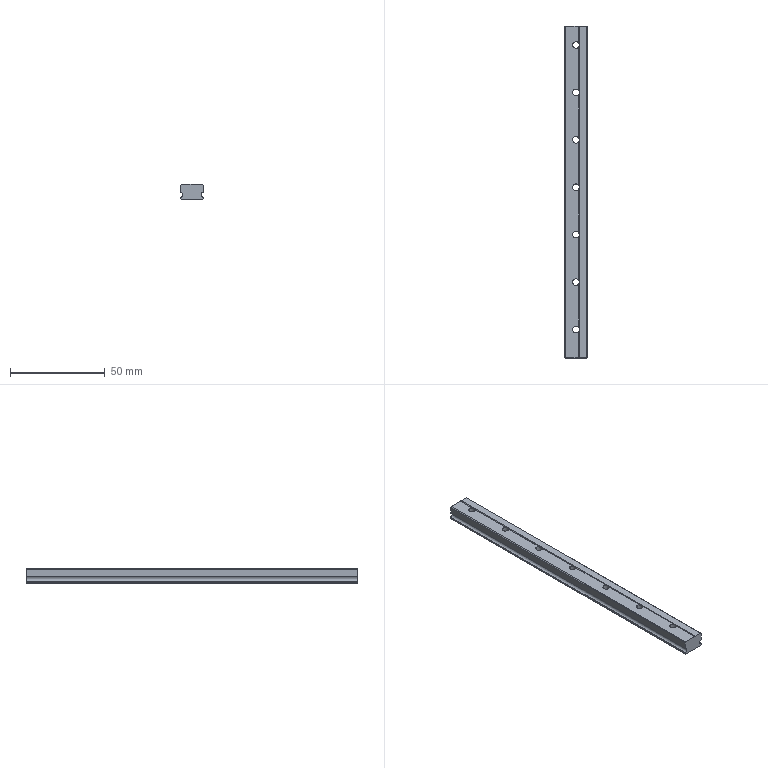Component | SolidWorks | MGN12H1R175Z0CGuideRailAssembly-1_MGN12HGuideRail-1 | 1 solid | 52 faces | box 12 x 175 x 8 mm | volume 14866 mm3 | cylinder 32 | plane 20 | commonest cylinder face diameters 6 x14 3.5 x14 2.5 x3 0.6 x1 | material 6061 Alloy
build123d program:
from build123d import *

# Parameters (mm, degrees)
SKETCH1_W                                            = 12
SKETCH1_H                                            = 175
BOSS_EXTRUDE1_DEPTH                                  = 8
F_2_5_2_5_DIAMETER_HOLE1_D                           = 2.5
F_0_6_0_6_DIAMETER_HOLE1_D                           = 0.6
CYLINDRICAL_COUNTERSUNK_HOLE_1_FOR_M3_HE_D           = 3.5
CYLINDRICAL_COUNTERSUNK_HOLE_1_FOR_M3_HE_CBORE_D     = 6
CYLINDRICAL_COUNTERSUNK_HOLE_1_FOR_M3_HE_CBORE_DEPTH = 3.5
CHAMFER1_SIZE                                        = 0.4
LPATTERN1_COUNT                                      = 7
LPATTERN1_PITCH                                      = 25


with BuildPart() as part:
    # Sketch1 → Boss-Extrude1 (new body)
    with BuildSketch(Plane.XZ):
        Rectangle(SKETCH1_W, SKETCH1_H)
    extrude(amount=-BOSS_EXTRUDE1_DEPTH)

    # 2.5 _2.5_ Diameter Hole1 (through all)
    with Locations(Plane(origin=(0, 0, -87.5), x_dir=(-1, 0, 0), z_dir=(0, 0, -1))):
        with Locations((-6, 5.5), (6, 5.5)):
            Hole(F_2_5_2_5_DIAMETER_HOLE1_D / 2)

    # 0.6 _0.6_ Diameter Hole1 (through all)
    with Locations(Plane.XY.offset(87.5)):
        with Locations((1.5, 0)):
            Hole(F_0_6_0_6_DIAMETER_HOLE1_D / 2)

    # Cylindrical Countersunk Hole 1 for M3 He (through all)
    with Locations(Plane(origin=(0, 8, 0), x_dir=(1, 0, 0), z_dir=(0, 1, 0))):
        with Locations((0, -77.5)):
            cylindrical_countersunk_hole_1_for_m3_he = CounterBoreHole(CYLINDRICAL_COUNTERSUNK_HOLE_1_FOR_M3_HE_D / 2, CYLINDRICAL_COUNTERSUNK_HOLE_1_FOR_M3_HE_CBORE_D / 2, CYLINDRICAL_COUNTERSUNK_HOLE_1_FOR_M3_HE_CBORE_DEPTH)

    # Chamfer1
    chamfer1_edges = [part.edges().sort_by_distance(p)[0] for p in [
        (-6, 8, 0),
        (6, 8, 0),
        (-6, 0, 0),
        (6, 0, 0),
    ]]
    chamfer(chamfer1_edges, length=CHAMFER1_SIZE)

    # LPattern1: Cylindrical Countersunk Hole 1 for M3 He ×7
    with Locations(*[(0, 0, -i * LPATTERN1_PITCH) for i in range(1, LPATTERN1_COUNT)]):
        add(cylindrical_countersunk_hole_1_for_m3_he, mode=Mode.SUBTRACT)


solid = part.part

# Placed as in the assembly
solid = solid.moved(Location((-24, 7.5, 0), (-90, 0, 0)))